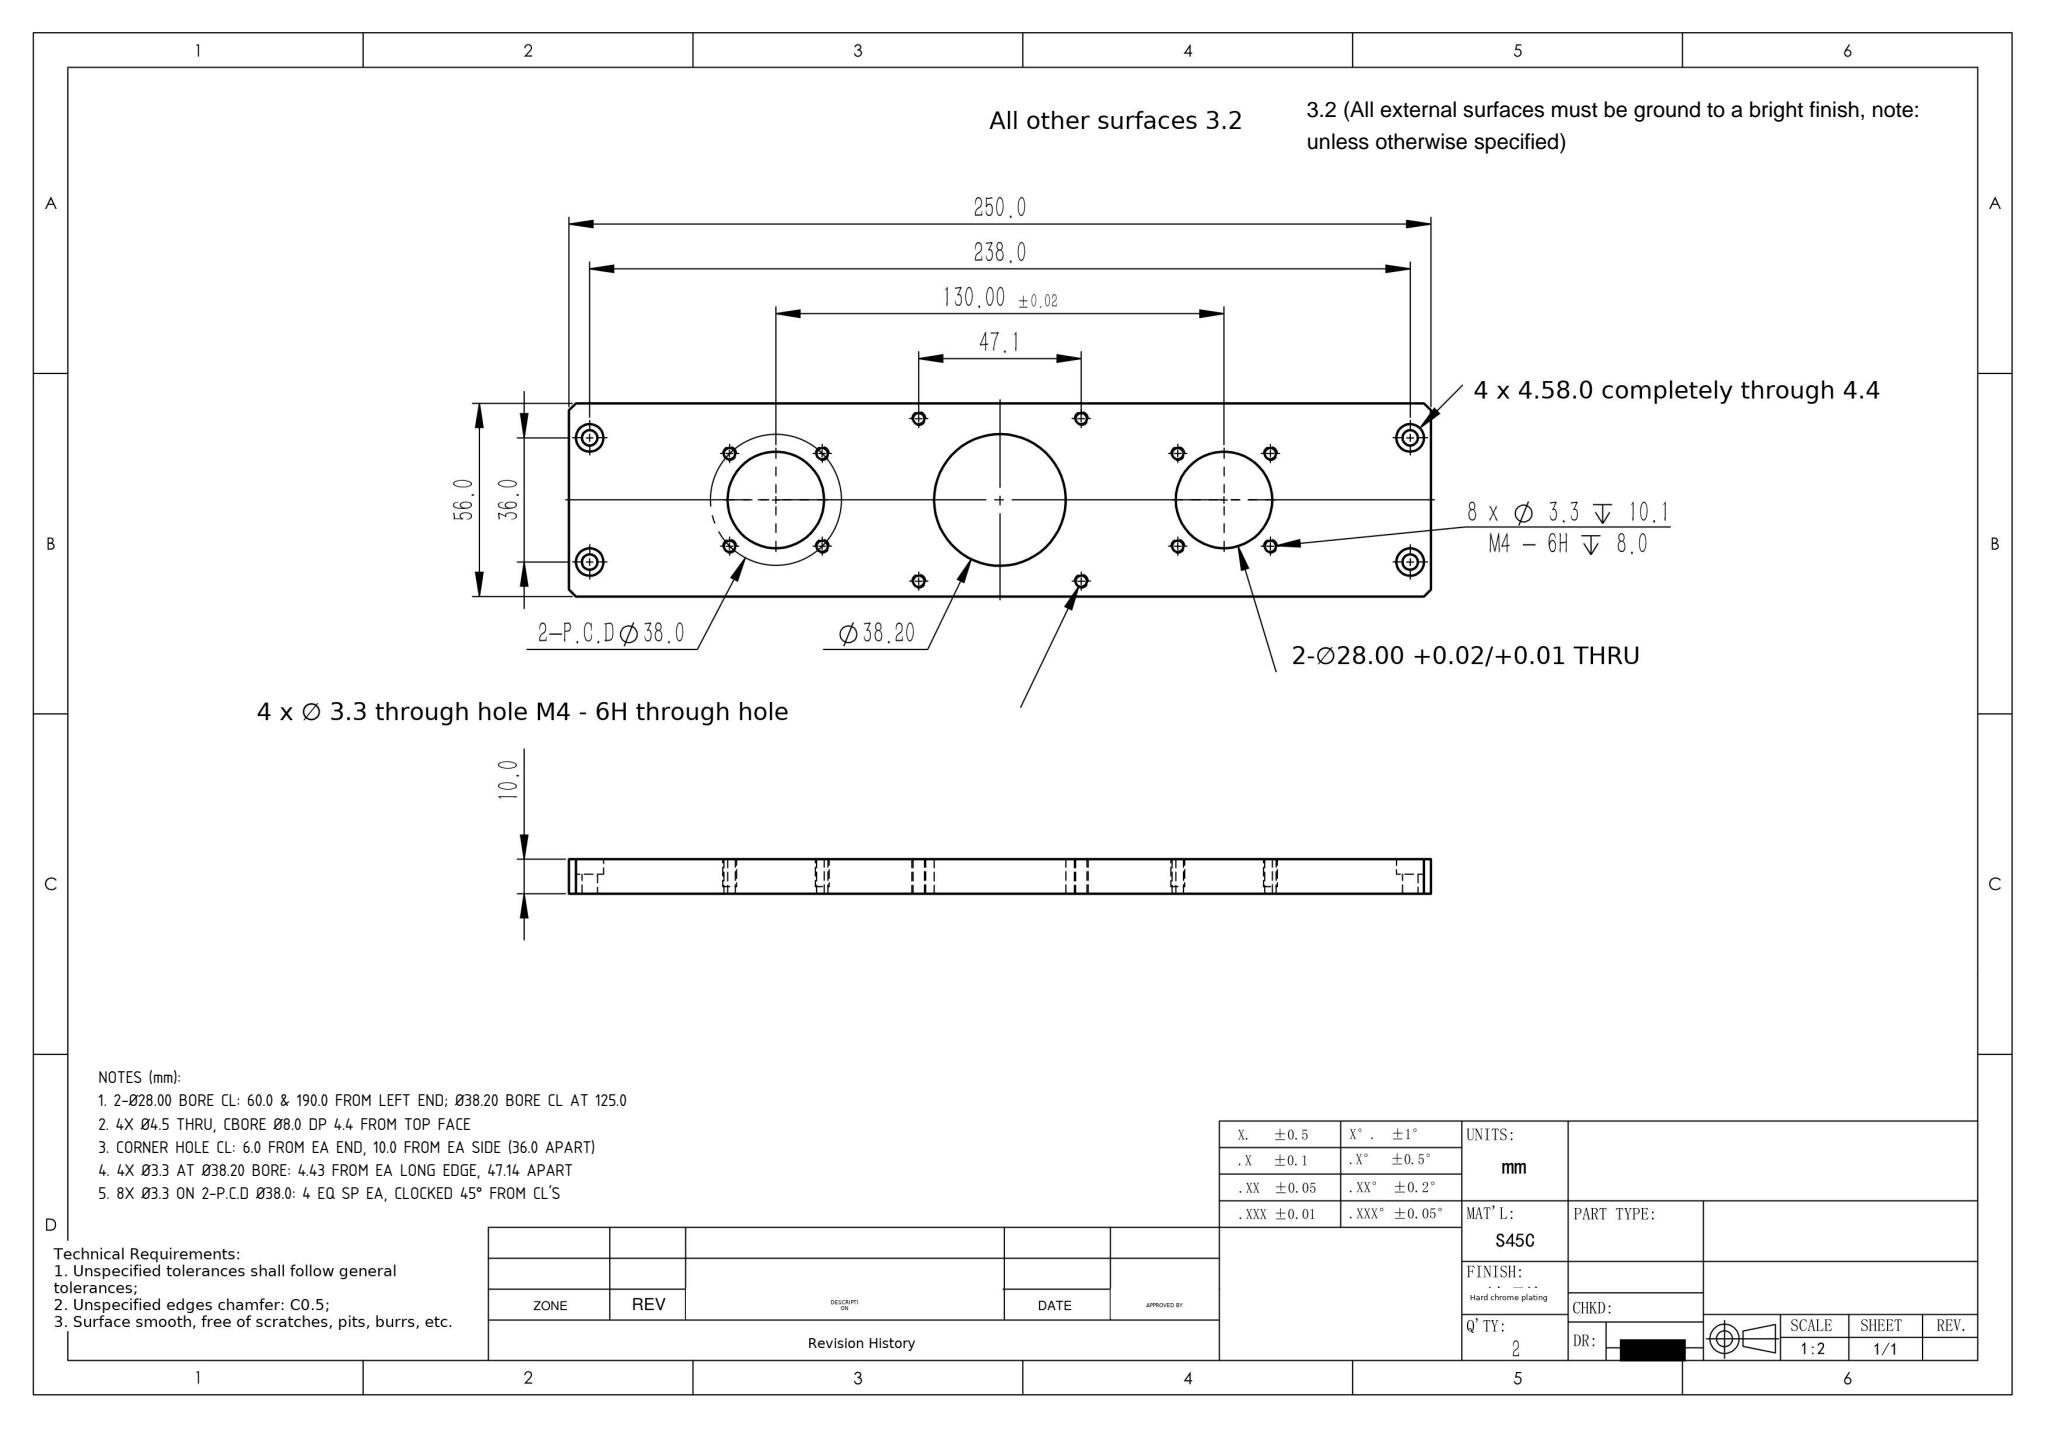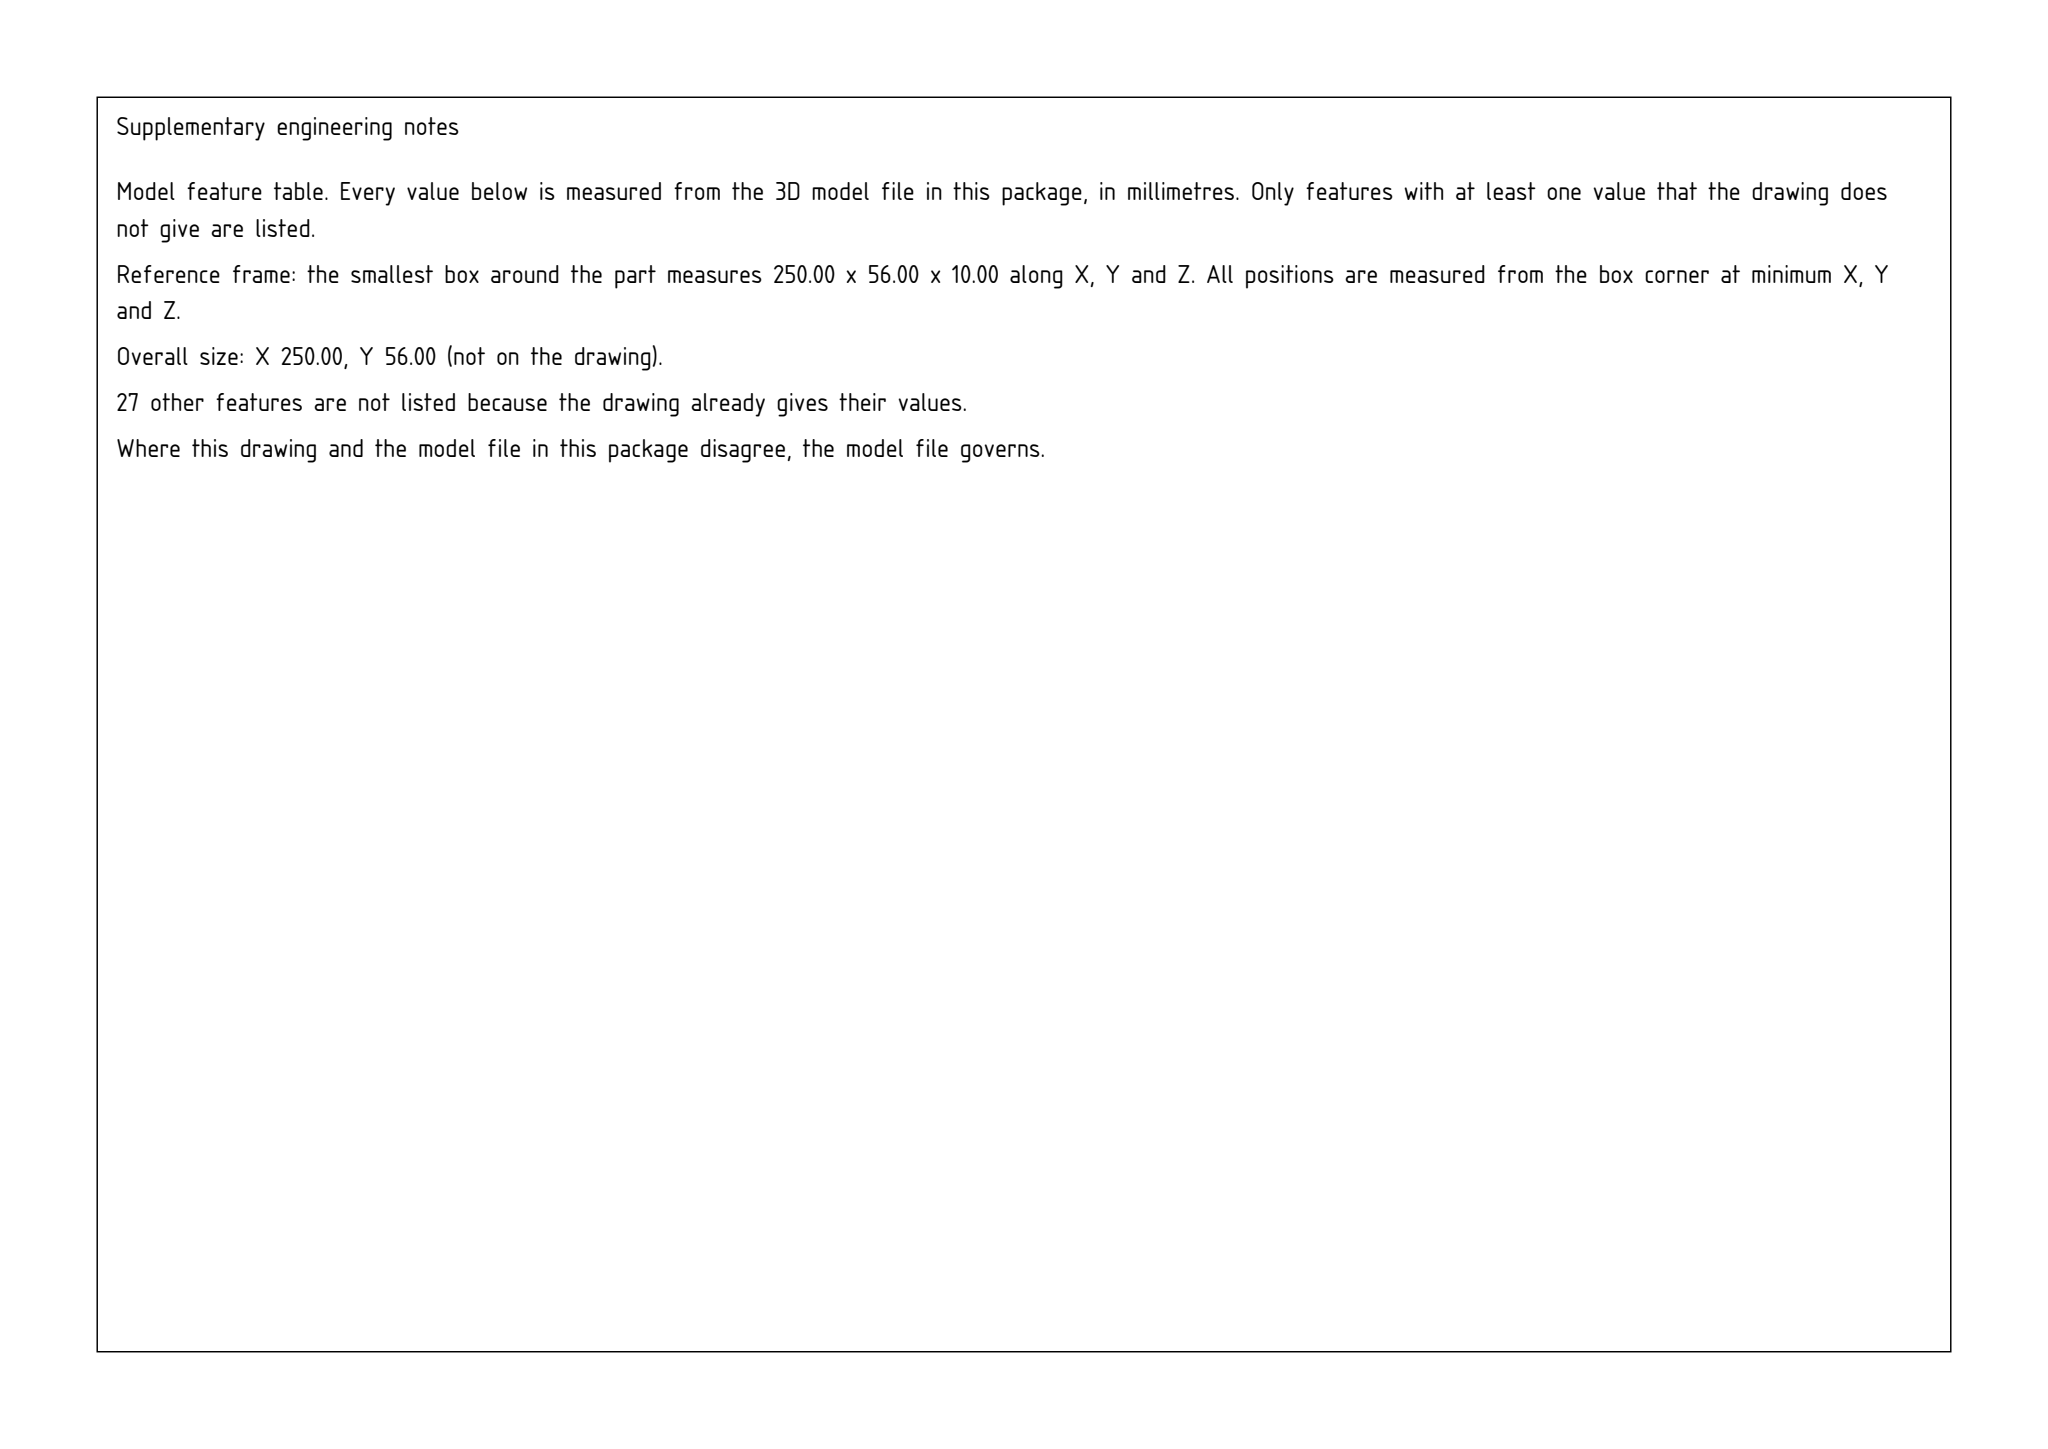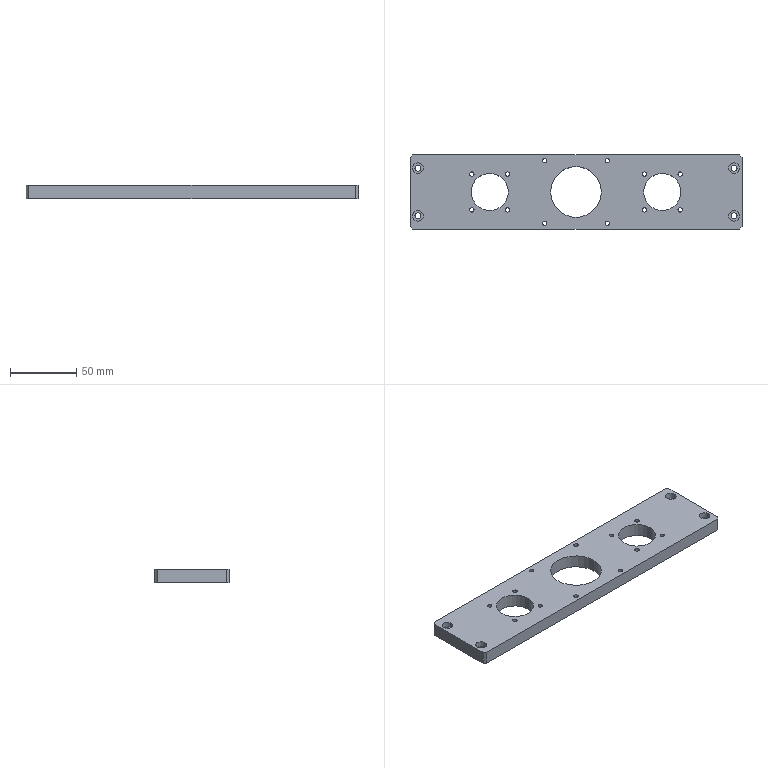Part | SolidWorks | mm | 1 solid | 60 faces | box 250 x 56 x 10 mm | volume 113877 mm3 | cylinder 46 | plane 14 | commonest cylinder face diameters 3.3 x24 8 x8 4.5 x8 28 x4 38.2 x2
Drawing notes:
2-Ø28.00 BORE CL: 60.0 & 190.0 FROM LEFT END; Ø38.20 BORE CL AT 125.0 | from the solid: Ø28 cyls at x=60.0 & 190.0, Ø38.2 at x=125.0, all y=28.0; bbox X=250.0
4X Ø4.5 THRU, CBORE Ø8.0 DP 4.4 FROM TOP FACE | from the solid: Ø4.5 L=5.6 coaxial w/ Ø8.0 L=4.4 at (6,10),(6,46),(244,10),(244,46); z-plane 5.6
CORNER HOLE CL: 6.0 FROM EA END, 10.0 FROM EA SIDE (36.0 APART) | from the solid: Ø4.5/Ø8.0 axes at x=6.0 & 244.0, y=10.0 & 46.0; bbox 250.0 x 56.0
4X Ø3.3 AT Ø38.20 BORE: 4.43 FROM EA LONG EDGE, 47.14 APART | from the solid: Ø3.3 at (101.43,4.43),(101.43,51.57),(148.57,4.43),(148.57,51.57); plate 56.0 wide
8X Ø3.3 ON 2-P.C.D Ø38.0: 4 EQ SP EA, CLOCKED 45° FROM CL'S | from the solid: Ø3.3 at (±13.44,±13.44) from bore CL 60,28 & 190,28 = R19.0 at 45°
build123d program:
from build123d import *

# Parameters (mm, degrees)
SKETCH1_W                                       = 250
SKETCH1_H                                       = 56
BOSS_EXTRUDE1_DEPTH                             = 10
SKETCH3_R                                       = 19.1
CUT_EXTRUDE2_DEPTH                              = 129.487
M4_TAPPED_HOLE2_D                               = 3.3
SKETCH8_R                                       = 14
CUT_EXTRUDE3_DEPTH                              = 129.487
M4_TAPPED_HOLE1_D                               = 3.3
M4_TAPPED_HOLE1_DEPTH                           = 10.1
M4_TAPPED_HOLE1_TIP                             = 0.9914
M4_HEX_SOCKET_HEAD_CAP_SCREW_CBORE1_D           = 4.5
M4_HEX_SOCKET_HEAD_CAP_SCREW_CBORE1_CBORE_D     = 8
M4_HEX_SOCKET_HEAD_CAP_SCREW_CBORE1_CBORE_DEPTH = 4.4
CHAMFER1_SIZE                                   = 2


with BuildPart() as part:
    # Sketch1 → Boss-Extrude1 (new body)
    with BuildSketch(Plane.XY):
        Rectangle(SKETCH1_W, SKETCH1_H)
    extrude(amount=BOSS_EXTRUDE1_DEPTH)

    # Sketch3 → Cut-Extrude2 (cut, through all)
    with BuildSketch(Plane(origin=(0, 0, 0), x_dir=(-1, 0, 0), z_dir=(0, 0, -1))):
        Circle(SKETCH3_R)
    extrude(amount=-CUT_EXTRUDE2_DEPTH, mode=Mode.SUBTRACT)

    # M4 Tapped Hole2 (through all)
    with Locations(Plane(origin=(0, 0, 0), x_dir=(-1, 0, 0), z_dir=(0, 0, -1))):
        with Locations((-23.57, -23.57), (-23.57, 23.57), (23.57, 23.57), (23.57, -23.57)):
            Hole(M4_TAPPED_HOLE2_D / 2)

    # Sketch8 → Cut-Extrude3 (cut, through all)
    with BuildSketch(Plane(origin=(0, 0, 0), x_dir=(-1, 0, 0), z_dir=(0, 0, -1))):
        with Locations((65, 0)):
            Circle(SKETCH8_R)
        with Locations((-65, 0)):
            Circle(SKETCH8_R)
    extrude(amount=-CUT_EXTRUDE3_DEPTH, mode=Mode.SUBTRACT)

    # M4 Tapped Hole1
    with Locations(Plane.XY.offset(10)):
        with Locations((-78.435, 13.435), (-51.565, 13.435), (-51.565, -13.435), (-78.435, -13.435), (51.565, -13.435), (78.435, -13.435), (78.435, 13.435), (51.565, 13.435)):
            Hole(M4_TAPPED_HOLE1_D / 2, depth=M4_TAPPED_HOLE1_DEPTH)
            with Locations((0, 0, -(M4_TAPPED_HOLE1_DEPTH + M4_TAPPED_HOLE1_TIP / 2))):  # 118° drill point
                Cone(0, M4_TAPPED_HOLE1_D / 2, M4_TAPPED_HOLE1_TIP, mode=Mode.SUBTRACT)

    # M4 Hex Socket Head Cap Screw CBORE1 (through all)
    with Locations(Plane.XY.offset(10)):
        with Locations((-119, 18), (-119, -18), (119, 18), (119, -18)):
            CounterBoreHole(M4_HEX_SOCKET_HEAD_CAP_SCREW_CBORE1_D / 2, M4_HEX_SOCKET_HEAD_CAP_SCREW_CBORE1_CBORE_D / 2, M4_HEX_SOCKET_HEAD_CAP_SCREW_CBORE1_CBORE_DEPTH)

    # Chamfer1
    chamfer1_edges = [part.edges().sort_by_distance(p)[0] for p in [
        (125, -28, 5),
        (-125, -28, 5),
        (-125, 28, 5),
        (125, 28, 5),
    ]]
    chamfer(chamfer1_edges, length=CHAMFER1_SIZE)


solid = part.part